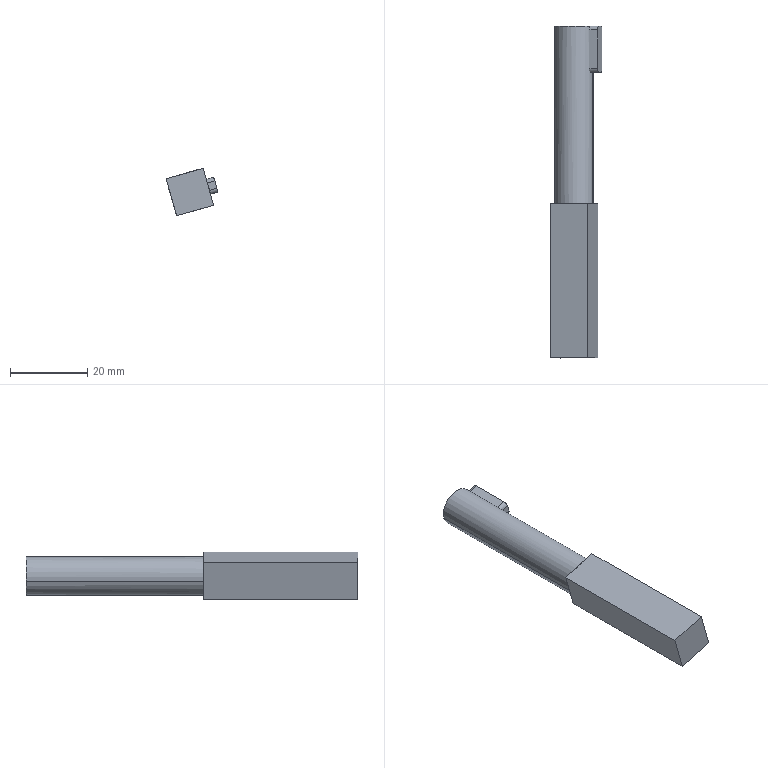Component | SolidWorks | DriveShaft2-2 | 1 solid | 20 faces | box 13.46 x 86 x 12.35 mm | volume 7713 mm3 | plane 14 | cylinder 6 | commonest cylinder face diameters 2 x4 10 x2
build123d program:
from build123d import *

# Parameters (mm, degrees)
SKETCH1_W                = 10
SKETCH1_H                = 10
BOSS_EXTRUDE1_DEPTH      = 40
SKETCH2_R                = 5
BOSS_EXTRUDE2_DEPTH      = 46
BOSS_EXTRUDE3_DEPTH      = 2
BOSS_EXTRUDE3_DEPTH_BACK = 6


with BuildPart() as part:
    # Sketch1 → Boss-Extrude1 (new body)
    with BuildSketch(Plane.XY):
        Rectangle(SKETCH1_W, SKETCH1_H)
    extrude(amount=BOSS_EXTRUDE1_DEPTH)

    # Sketch2 → Boss-Extrude2 (add)
    with BuildSketch(Plane(origin=(0, 0, 0), x_dir=(-1, 0, 0), z_dir=(0, 0, -1))):
        Circle(SKETCH2_R)
    extrude(amount=BOSS_EXTRUDE2_DEPTH)

    # Sketch3 → Boss-Extrude3 (add, two sides: drawn at the far end of the back side and taken through both)
    with BuildSketch(Plane(origin=(5, 0, 0), x_dir=(0, 0, -1), z_dir=(1, 0, 0)).offset(-BOSS_EXTRUDE3_DEPTH_BACK)):
        with BuildLine():
            Line((45, 2), (35, 2))
            ThreePointArc((35, 2), (34.293, 1.707), (34, 1))
            Line((34, 1), (34, -1))
            ThreePointArc((34, -1), (34.293, -1.707), (35, -2))
            Line((35, -2), (45, -2))
            ThreePointArc((45, -2), (45.707, -1.707), (46, -1))
            Line((46, -1), (46, 1))
            ThreePointArc((46, 1), (45.707, 1.707), (45, 2))
        make_face()
    extrude(amount=BOSS_EXTRUDE3_DEPTH + BOSS_EXTRUDE3_DEPTH_BACK)


solid = part.part

# Placed as in the assembly
solid = solid.moved(Location((-65.043, 476.747, 900.064), (90, 0, 15.845)))
STEP:
#1=COLOUR_RGB('',0.7922,0.8196,0.9333);
#2=FILL_AREA_STYLE_COLOUR('',#1);
#3=FILL_AREA_STYLE('',(#2));
#4=SURFACE_STYLE_FILL_AREA(#3);
#5=SURFACE_SIDE_STYLE('',(#4));
#6=SURFACE_STYLE_USAGE(.BOTH.,#5);
#7=PRESENTATION_STYLE_ASSIGNMENT((#6));
#8=CARTESIAN_POINT('',(-2.75,20.581,35.382));
#9=VERTEX_POINT('',#8);
#10=CARTESIAN_POINT('',(-2.386,20.581,35.526));
#11=VERTEX_POINT('',#10);
#12=CARTESIAN_POINT('',(-2.561,20.581,35.436));
#13=DIRECTION('',(-0.,1.,0.));
#14=DIRECTION('',(-0.962,0.,-0.273));
#15=AXIS2_PLACEMENT_3D('',#12,#13,#14);
#16=CIRCLE('',#15,0.1969);
#17=EDGE_CURVE('',#9,#11,#16,.T.);
#18=ORIENTED_EDGE('',*,*,#17,.F.);
#19=CARTESIAN_POINT('',(-2.75,18.77,35.382));
#20=VERTEX_POINT('',#19);
#21=CARTESIAN_POINT('',(-2.75,20.581,35.382));
#22=DIRECTION('',(0.,-1.,-0.));
#23=VECTOR('',#22,39.37);
#24=LINE('',#21,#23);
#25=EDGE_CURVE('',#9,#20,#24,.T.);
#26=ORIENTED_EDGE('',*,*,#25,.T.);
#27=CARTESIAN_POINT('',(-2.615,18.77,35.625));
#28=VERTEX_POINT('',#27);
#29=CARTESIAN_POINT('',(-2.561,18.77,35.436));
#30=DIRECTION('',(-0.,1.,0.));
#31=DIRECTION('',(-0.962,0.,-0.273));
#32=AXIS2_PLACEMENT_3D('',#29,#30,#31);
#33=CIRCLE('',#32,0.1969);
#34=EDGE_CURVE('',#20,#28,#33,.T.);
#35=ORIENTED_EDGE('',*,*,#34,.T.);
#36=CARTESIAN_POINT('',(-2.371,18.77,35.489));
#37=VERTEX_POINT('',#36);
#38=CARTESIAN_POINT('',(-2.561,18.77,35.436));
#39=DIRECTION('',(-0.,1.,0.));
#40=DIRECTION('',(-0.962,0.,-0.273));
#41=AXIS2_PLACEMENT_3D('',#38,#39,#40);
#42=CIRCLE('',#41,0.1969);
#43=EDGE_CURVE('',#28,#37,#42,.T.);
#44=ORIENTED_EDGE('',*,*,#43,.T.);
#45=CARTESIAN_POINT('',(-2.371,20.108,35.489));
#46=VERTEX_POINT('',#45);
#47=CARTESIAN_POINT('',(-2.371,20.581,35.489));
#48=DIRECTION('',(0.,-1.,-0.));
#49=VECTOR('',#48,39.37);
#50=LINE('',#47,#49);
#51=EDGE_CURVE('',#46,#37,#50,.T.);
#52=ORIENTED_EDGE('',*,*,#51,.F.);
#53=CARTESIAN_POINT('',(-2.386,20.108,35.526));
#54=VERTEX_POINT('',#53);
#55=CARTESIAN_POINT('',(-2.561,20.108,35.436));
#56=DIRECTION('',(0.,-1.,-0.));
#57=DIRECTION('',(0.962,0.,0.273));
#58=AXIS2_PLACEMENT_3D('',#55,#56,#57);
#59=CIRCLE('',#58,0.1969);
#60=EDGE_CURVE('',#46,#54,#59,.T.);
#61=ORIENTED_EDGE('',*,*,#60,.T.);
#62=CARTESIAN_POINT('',(-2.409,20.148,35.561));
#63=VERTEX_POINT('',#62);
#64=CARTESIAN_POINT('',(-2.386,20.108,35.526));
#65=CARTESIAN_POINT('',(-2.388,20.108,35.531));
#66=CARTESIAN_POINT('',(-2.391,20.109,35.535));
#67=CARTESIAN_POINT('',(-2.396,20.113,35.544));
#68=CARTESIAN_POINT('',(-2.399,20.116,35.547));
#69=CARTESIAN_POINT('',(-2.403,20.123,35.554));
#70=CARTESIAN_POINT('',(-2.405,20.127,35.556));
#71=CARTESIAN_POINT('',(-2.408,20.137,35.56));
#72=CARTESIAN_POINT('',(-2.409,20.142,35.561));
#73=CARTESIAN_POINT('',(-2.409,20.148,35.561));
#74=B_SPLINE_CURVE_WITH_KNOTS('',3,(#64,#65,#66,#67,#68,#69,#70,#71,#72,#73),.UNSPECIFIED.,.F.,.F.,(4,2,2,2,4),(0.00157,0.00197,0.00237,0.002769,0.003169),.UNSPECIFIED.);
#75=EDGE_CURVE('',#54,#63,#74,.T.);
#76=ORIENTED_EDGE('',*,*,#75,.T.);
#77=CARTESIAN_POINT('',(-2.409,20.541,35.561));
#78=VERTEX_POINT('',#77);
#79=CARTESIAN_POINT('',(-2.409,20.581,35.561));
#80=DIRECTION('',(-0.,1.,0.));
#81=VECTOR('',#80,39.37);
#82=LINE('',#79,#81);
#83=EDGE_CURVE('',#63,#78,#82,.T.);
#84=ORIENTED_EDGE('',*,*,#83,.T.);
#85=CARTESIAN_POINT('',(-2.386,20.581,35.526));
#86=CARTESIAN_POINT('',(-2.388,20.581,35.531));
#87=CARTESIAN_POINT('',(-2.391,20.58,35.535));
#88=CARTESIAN_POINT('',(-2.396,20.576,35.544));
#89=CARTESIAN_POINT('',(-2.399,20.573,35.547));
#90=CARTESIAN_POINT('',(-2.403,20.566,35.554));
#91=CARTESIAN_POINT('',(-2.405,20.561,35.556));
#92=CARTESIAN_POINT('',(-2.408,20.552,35.56));
#93=CARTESIAN_POINT('',(-2.409,20.547,35.561));
#94=CARTESIAN_POINT('',(-2.409,20.541,35.561));
#95=B_SPLINE_CURVE_WITH_KNOTS('',3,(#85,#86,#87,#88,#89,#90,#91,#92,#93,#94),.UNSPECIFIED.,.F.,.F.,(4,2,2,2,4),(0.,0.0003995,0.0007989,0.001198,0.001598),.UNSPECIFIED.);
#96=EDGE_CURVE('',#11,#78,#95,.T.);
#97=ORIENTED_EDGE('',*,*,#96,.F.);
#98=EDGE_LOOP('',(#18,#26,#35,#44,#52,#61,#76,#84,#97));
#99=FACE_OUTER_BOUND('',#98,.T.);
#100=CARTESIAN_POINT('',(-2.561,20.581,35.436));
#101=DIRECTION('',(0.,-1.,-0.));
#102=DIRECTION('',(0.962,0.,0.273));
#103=AXIS2_PLACEMENT_3D('',#100,#101,#102);
#104=CYLINDRICAL_SURFACE('',#103,0.1969);
#105=ADVANCED_FACE('',(#99),#104,.T.);
#106=ORIENTED_EDGE('',*,*,#25,.F.);
#107=CARTESIAN_POINT('',(-2.364,20.581,35.45));
#108=VERTEX_POINT('',#107);
#109=CARTESIAN_POINT('',(-2.561,20.581,35.436));
#110=DIRECTION('',(-0.,1.,0.));
#111=DIRECTION('',(-0.962,0.,-0.273));
#112=AXIS2_PLACEMENT_3D('',#109,#110,#111);
#113=CIRCLE('',#112,0.1969);
#114=EDGE_CURVE('',#108,#9,#113,.T.);
#115=ORIENTED_EDGE('',*,*,#114,.F.);
#116=CARTESIAN_POINT('',(-2.366,20.541,35.409));
#117=VERTEX_POINT('',#116);
#118=CARTESIAN_POINT('',(-2.364,20.581,35.45));
#119=CARTESIAN_POINT('',(-2.364,20.581,35.445));
#120=CARTESIAN_POINT('',(-2.364,20.58,35.44));
#121=CARTESIAN_POINT('',(-2.364,20.576,35.43));
#122=CARTESIAN_POINT('',(-2.364,20.573,35.425));
#123=CARTESIAN_POINT('',(-2.365,20.566,35.418));
#124=CARTESIAN_POINT('',(-2.365,20.561,35.415));
#125=CARTESIAN_POINT('',(-2.366,20.552,35.41));
#126=CARTESIAN_POINT('',(-2.366,20.546,35.409));
#127=CARTESIAN_POINT('',(-2.366,20.541,35.409));
#128=B_SPLINE_CURVE_WITH_KNOTS('',3,(#118,#119,#120,#121,#122,#123,#124,#125,#126,#127),.UNSPECIFIED.,.F.,.F.,(4,2,2,2,4),(0.,0.0003998,0.0007997,0.001199,0.001599),.UNSPECIFIED.);
#129=EDGE_CURVE('',#108,#117,#128,.T.);
#130=ORIENTED_EDGE('',*,*,#129,.T.);
#131=CARTESIAN_POINT('',(-2.366,20.148,35.409));
#132=VERTEX_POINT('',#131);
#133=CARTESIAN_POINT('',(-2.366,20.581,35.409));
#134=DIRECTION('',(0.,-1.,-0.));
#135=VECTOR('',#134,39.37);
#136=LINE('',#133,#135);
#137=EDGE_CURVE('',#117,#132,#136,.T.);
#138=ORIENTED_EDGE('',*,*,#137,.T.);
#139=CARTESIAN_POINT('',(-2.364,20.108,35.45));
#140=VERTEX_POINT('',#139);
#141=CARTESIAN_POINT('',(-2.366,20.148,35.409));
#142=CARTESIAN_POINT('',(-2.366,20.142,35.409));
#143=CARTESIAN_POINT('',(-2.366,20.137,35.41));
#144=CARTESIAN_POINT('',(-2.365,20.127,35.415));
#145=CARTESIAN_POINT('',(-2.365,20.123,35.418));
#146=CARTESIAN_POINT('',(-2.364,20.112,35.429));
#147=CARTESIAN_POINT('',(-2.364,20.108,35.44));
#148=CARTESIAN_POINT('',(-2.364,20.108,35.45));
#149=B_SPLINE_CURVE_WITH_KNOTS('',3,(#141,#142,#143,#144,#145,#146,#147,#148),.UNSPECIFIED.,.F.,.F.,(4,2,2,4),(0.003169,0.003569,0.003968,0.004767),.UNSPECIFIED.);
#150=EDGE_CURVE('',#132,#140,#149,.T.);
#151=ORIENTED_EDGE('',*,*,#150,.T.);
#152=CARTESIAN_POINT('',(-2.561,20.108,35.436));
#153=DIRECTION('',(0.,-1.,-0.));
#154=DIRECTION('',(0.962,0.,0.273));
#155=AXIS2_PLACEMENT_3D('',#152,#153,#154);
#156=CIRCLE('',#155,0.1969);
#157=EDGE_CURVE('',#140,#46,#156,.T.);
#158=ORIENTED_EDGE('',*,*,#157,.T.);
#159=ORIENTED_EDGE('',*,*,#51,.T.);
#160=CARTESIAN_POINT('',(-2.507,18.77,35.246));
#161=VERTEX_POINT('',#160);
#162=CARTESIAN_POINT('',(-2.561,18.77,35.436));
#163=DIRECTION('',(-0.,1.,0.));
#164=DIRECTION('',(-0.962,0.,-0.273));
#165=AXIS2_PLACEMENT_3D('',#162,#163,#164);
#166=CIRCLE('',#165,0.1969);
#167=EDGE_CURVE('',#37,#161,#166,.T.);
#168=ORIENTED_EDGE('',*,*,#167,.T.);
#169=CARTESIAN_POINT('',(-2.561,18.77,35.436));
#170=DIRECTION('',(-0.,1.,0.));
#171=DIRECTION('',(-0.962,0.,-0.273));
#172=AXIS2_PLACEMENT_3D('',#169,#170,#171);
#173=CIRCLE('',#172,0.1969);
#174=EDGE_CURVE('',#161,#20,#173,.T.);
#175=ORIENTED_EDGE('',*,*,#174,.T.);
#176=EDGE_LOOP('',(#106,#115,#130,#138,#151,#158,#159,#168,#175));
#177=FACE_OUTER_BOUND('',#176,.T.);
#178=CARTESIAN_POINT('',(-2.561,20.581,35.436));
#179=DIRECTION('',(0.,-1.,-0.));
#180=DIRECTION('',(0.962,0.,0.273));
#181=AXIS2_PLACEMENT_3D('',#178,#179,#180);
#182=CYLINDRICAL_SURFACE('',#181,0.1969);
#183=ADVANCED_FACE('',(#177),#182,.T.);
#184=ORIENTED_EDGE('',*,*,#34,.F.);
#185=CARTESIAN_POINT('',(-2.804,18.77,35.571));
#186=VERTEX_POINT('',#185);
#187=CARTESIAN_POINT('',(-2.696,18.77,35.192));
#188=DIRECTION('',(0.273,0.,-0.962));
#189=VECTOR('',#188,39.37);
#190=LINE('',#187,#189);
#191=EDGE_CURVE('',#186,#20,#190,.T.);
#192=ORIENTED_EDGE('',*,*,#191,.F.);
#193=CARTESIAN_POINT('',(-2.804,18.77,35.571));
#194=DIRECTION('',(-0.962,-0.,-0.273));
#195=VECTOR('',#194,39.37);
#196=LINE('',#193,#195);
#197=EDGE_CURVE('',#28,#186,#196,.T.);
#198=ORIENTED_EDGE('',*,*,#197,.F.);
#199=EDGE_LOOP('',(#184,#192,#198));
#200=FACE_OUTER_BOUND('',#199,.T.);
#201=CARTESIAN_POINT('',(-2.561,18.77,35.436));
#202=DIRECTION('',(-0.,1.,0.));
#203=DIRECTION('',(-0.962,-0.,-0.273));
#204=AXIS2_PLACEMENT_3D('',#201,#202,#203);
#205=PLANE('',#204);
#206=ADVANCED_FACE('',(#200),#205,.T.);
#207=ORIENTED_EDGE('',*,*,#43,.F.);
#208=CARTESIAN_POINT('',(-2.425,18.77,35.679));
#209=VERTEX_POINT('',#208);
#210=CARTESIAN_POINT('',(-2.804,18.77,35.571));
#211=DIRECTION('',(-0.962,-0.,-0.273));
#212=VECTOR('',#211,39.37);
#213=LINE('',#210,#212);
#214=EDGE_CURVE('',#209,#28,#213,.T.);
#215=ORIENTED_EDGE('',*,*,#214,.F.);
#216=CARTESIAN_POINT('',(-2.318,18.77,35.3));
#217=DIRECTION('',(-0.273,-0.,0.962));
#218=VECTOR('',#217,39.37);
#219=LINE('',#216,#218);
#220=EDGE_CURVE('',#37,#209,#219,.T.);
#221=ORIENTED_EDGE('',*,*,#220,.F.);
#222=EDGE_LOOP('',(#207,#215,#221));
#223=FACE_OUTER_BOUND('',#222,.T.);
#224=CARTESIAN_POINT('',(-2.561,18.77,35.436));
#225=DIRECTION('',(-0.,1.,0.));
#226=DIRECTION('',(-0.962,-0.,-0.273));
#227=AXIS2_PLACEMENT_3D('',#224,#225,#226);
#228=PLANE('',#227);
#229=ADVANCED_FACE('',(#223),#228,.T.);
#230=ORIENTED_EDGE('',*,*,#167,.F.);
#231=CARTESIAN_POINT('',(-2.318,18.77,35.3));
#232=VERTEX_POINT('',#231);
#233=CARTESIAN_POINT('',(-2.318,18.77,35.3));
#234=DIRECTION('',(-0.273,-0.,0.962));
#235=VECTOR('',#234,39.37);
#236=LINE('',#233,#235);
#237=EDGE_CURVE('',#232,#37,#236,.T.);
#238=ORIENTED_EDGE('',*,*,#237,.F.);
#239=CARTESIAN_POINT('',(-2.696,18.77,35.192));
#240=DIRECTION('',(0.962,0.,0.273));
#241=VECTOR('',#240,39.37);
#242=LINE('',#239,#241);
#243=EDGE_CURVE('',#161,#232,#242,.T.);
#244=ORIENTED_EDGE('',*,*,#243,.F.);
#245=EDGE_LOOP('',(#230,#238,#244));
#246=FACE_OUTER_BOUND('',#245,.T.);
#247=CARTESIAN_POINT('',(-2.561,18.77,35.436));
#248=DIRECTION('',(-0.,1.,0.));
#249=DIRECTION('',(-0.962,-0.,-0.273));
#250=AXIS2_PLACEMENT_3D('',#247,#248,#249);
#251=PLANE('',#250);
#252=ADVANCED_FACE('',(#246),#251,.T.);
#253=ORIENTED_EDGE('',*,*,#237,.T.);
#254=ORIENTED_EDGE('',*,*,#220,.T.);
#255=CARTESIAN_POINT('',(-2.425,17.195,35.679));
#256=VERTEX_POINT('',#255);
#257=CARTESIAN_POINT('',(-2.425,17.195,35.679));
#258=DIRECTION('',(-0.,1.,0.));
#259=VECTOR('',#258,39.37);
#260=LINE('',#257,#259);
#261=EDGE_CURVE('',#256,#209,#260,.T.);
#262=ORIENTED_EDGE('',*,*,#261,.F.);
#263=CARTESIAN_POINT('',(-2.318,17.195,35.3));
#264=VERTEX_POINT('',#263);
#265=CARTESIAN_POINT('',(-2.318,17.195,35.3));
#266=DIRECTION('',(-0.273,-0.,0.962));
#267=VECTOR('',#266,39.37);
#268=LINE('',#265,#267);
#269=EDGE_CURVE('',#264,#256,#268,.T.);
#270=ORIENTED_EDGE('',*,*,#269,.F.);
#271=CARTESIAN_POINT('',(-2.318,17.195,35.3));
#272=DIRECTION('',(-0.,1.,0.));
#273=VECTOR('',#272,39.37);
#274=LINE('',#271,#273);
#275=EDGE_CURVE('',#264,#232,#274,.T.);
#276=ORIENTED_EDGE('',*,*,#275,.T.);
#277=EDGE_LOOP('',(#253,#254,#262,#270,#276));
#278=FACE_OUTER_BOUND('',#277,.T.);
#279=CARTESIAN_POINT('',(-2.318,17.195,35.3));
#280=DIRECTION('',(-0.962,-0.,-0.273));
#281=DIRECTION('',(0.,-1.,-0.));
#282=AXIS2_PLACEMENT_3D('',#279,#280,#281);
#283=PLANE('',#282);
#284=ADVANCED_FACE('',(#278),#283,.F.);
#285=ORIENTED_EDGE('',*,*,#214,.T.);
#286=ORIENTED_EDGE('',*,*,#197,.T.);
#287=CARTESIAN_POINT('',(-2.804,17.195,35.571));
#288=VERTEX_POINT('',#287);
#289=CARTESIAN_POINT('',(-2.804,17.195,35.571));
#290=DIRECTION('',(-0.,1.,0.));
#291=VECTOR('',#290,39.37);
#292=LINE('',#289,#291);
#293=EDGE_CURVE('',#288,#186,#292,.T.);
#294=ORIENTED_EDGE('',*,*,#293,.F.);
#295=CARTESIAN_POINT('',(-2.804,17.195,35.571));
#296=DIRECTION('',(-0.962,-0.,-0.273));
#297=VECTOR('',#296,39.37);
#298=LINE('',#295,#297);
#299=EDGE_CURVE('',#256,#288,#298,.T.);
#300=ORIENTED_EDGE('',*,*,#299,.F.);
#301=ORIENTED_EDGE('',*,*,#261,.T.);
#302=EDGE_LOOP('',(#285,#286,#294,#300,#301));
#303=FACE_OUTER_BOUND('',#302,.T.);
#304=CARTESIAN_POINT('',(-2.804,17.195,35.571));
#305=DIRECTION('',(0.273,0.,-0.962));
#306=DIRECTION('',(-0.,1.,0.));
#307=AXIS2_PLACEMENT_3D('',#304,#305,#306);
#308=PLANE('',#307);
#309=ADVANCED_FACE('',(#303),#308,.F.);
#310=ORIENTED_EDGE('',*,*,#191,.T.);
#311=CARTESIAN_POINT('',(-2.696,18.77,35.192));
#312=VERTEX_POINT('',#311);
#313=CARTESIAN_POINT('',(-2.696,18.77,35.192));
#314=DIRECTION('',(0.273,0.,-0.962));
#315=VECTOR('',#314,39.37);
#316=LINE('',#313,#315);
#317=EDGE_CURVE('',#20,#312,#316,.T.);
#318=ORIENTED_EDGE('',*,*,#317,.T.);
#319=CARTESIAN_POINT('',(-2.696,17.195,35.192));
#320=VERTEX_POINT('',#319);
#321=CARTESIAN_POINT('',(-2.696,17.195,35.192));
#322=DIRECTION('',(-0.,1.,0.));
#323=VECTOR('',#322,39.37);
#324=LINE('',#321,#323);
#325=EDGE_CURVE('',#320,#312,#324,.T.);
#326=ORIENTED_EDGE('',*,*,#325,.F.);
#327=CARTESIAN_POINT('',(-2.696,17.195,35.192));
#328=DIRECTION('',(0.273,0.,-0.962));
#329=VECTOR('',#328,39.37);
#330=LINE('',#327,#329);
#331=EDGE_CURVE('',#288,#320,#330,.T.);
#332=ORIENTED_EDGE('',*,*,#331,.F.);
#333=ORIENTED_EDGE('',*,*,#293,.T.);
#334=EDGE_LOOP('',(#310,#318,#326,#332,#333));
#335=FACE_OUTER_BOUND('',#334,.T.);
#336=CARTESIAN_POINT('',(-2.696,17.195,35.192));
#337=DIRECTION('',(0.962,0.,0.273));
#338=DIRECTION('',(-0.,1.,0.));
#339=AXIS2_PLACEMENT_3D('',#336,#337,#338);
#340=PLANE('',#339);
#341=ADVANCED_FACE('',(#335),#340,.F.);
#342=CARTESIAN_POINT('',(-2.696,18.77,35.192));
#343=DIRECTION('',(0.962,0.,0.273));
#344=VECTOR('',#343,39.37);
#345=LINE('',#342,#344);
#346=EDGE_CURVE('',#312,#161,#345,.T.);
#347=ORIENTED_EDGE('',*,*,#346,.T.);
#348=ORIENTED_EDGE('',*,*,#243,.T.);
#349=ORIENTED_EDGE('',*,*,#275,.F.);
#350=CARTESIAN_POINT('',(-2.696,17.195,35.192));
#351=DIRECTION('',(0.962,0.,0.273));
#352=VECTOR('',#351,39.37);
#353=LINE('',#350,#352);
#354=EDGE_CURVE('',#320,#264,#353,.T.);
#355=ORIENTED_EDGE('',*,*,#354,.F.);
#356=ORIENTED_EDGE('',*,*,#325,.T.);
#357=EDGE_LOOP('',(#347,#348,#349,#355,#356));
#358=FACE_OUTER_BOUND('',#357,.T.);
#359=CARTESIAN_POINT('',(-2.696,17.195,35.192));
#360=DIRECTION('',(-0.273,-0.,0.962));
#361=DIRECTION('',(0.,-1.,-0.));
#362=AXIS2_PLACEMENT_3D('',#359,#360,#361);
#363=PLANE('',#362);
#364=ADVANCED_FACE('',(#358),#363,.F.);
#365=ORIENTED_EDGE('',*,*,#269,.T.);
#366=ORIENTED_EDGE('',*,*,#299,.T.);
#367=ORIENTED_EDGE('',*,*,#331,.T.);
#368=ORIENTED_EDGE('',*,*,#354,.T.);
#369=EDGE_LOOP('',(#365,#366,#367,#368));
#370=FACE_OUTER_BOUND('',#369,.T.);
#371=CARTESIAN_POINT('',(-2.561,17.195,35.436));
#372=DIRECTION('',(-0.,1.,0.));
#373=DIRECTION('',(-0.962,-0.,-0.273));
#374=AXIS2_PLACEMENT_3D('',#371,#372,#373);
#375=PLANE('',#374);
#376=ADVANCED_FACE('',(#370),#375,.F.);
#377=ORIENTED_EDGE('',*,*,#174,.F.);
#378=ORIENTED_EDGE('',*,*,#346,.F.);
#379=ORIENTED_EDGE('',*,*,#317,.F.);
#380=EDGE_LOOP('',(#377,#378,#379));
#381=FACE_OUTER_BOUND('',#380,.T.);
#382=CARTESIAN_POINT('',(-2.561,18.77,35.436));
#383=DIRECTION('',(-0.,1.,0.));
#384=DIRECTION('',(-0.962,-0.,-0.273));
#385=AXIS2_PLACEMENT_3D('',#382,#383,#384);
#386=PLANE('',#385);
#387=ADVANCED_FACE('',(#381),#386,.T.);
#388=ORIENTED_EDGE('',*,*,#114,.T.);
#389=ORIENTED_EDGE('',*,*,#17,.T.);
#390=CARTESIAN_POINT('',(-2.306,20.581,35.549));
#391=VERTEX_POINT('',#390);
#392=CARTESIAN_POINT('',(-2.609,20.581,35.463));
#393=DIRECTION('',(0.962,0.,0.273));
#394=VECTOR('',#393,39.37);
#395=LINE('',#392,#394);
#396=EDGE_CURVE('',#11,#391,#395,.T.);
#397=ORIENTED_EDGE('',*,*,#396,.T.);
#398=CARTESIAN_POINT('',(-2.285,20.581,35.473));
#399=VERTEX_POINT('',#398);
#400=CARTESIAN_POINT('',(-2.285,20.581,35.473));
#401=DIRECTION('',(-0.273,-0.,0.962));
#402=VECTOR('',#401,39.37);
#403=LINE('',#400,#402);
#404=EDGE_CURVE('',#399,#391,#403,.T.);
#405=ORIENTED_EDGE('',*,*,#404,.F.);
#406=CARTESIAN_POINT('',(-2.588,20.581,35.387));
#407=DIRECTION('',(0.962,0.,0.273));
#408=VECTOR('',#407,39.37);
#409=LINE('',#406,#408);
#410=EDGE_CURVE('',#108,#399,#409,.T.);
#411=ORIENTED_EDGE('',*,*,#410,.F.);
#412=EDGE_LOOP('',(#388,#389,#397,#405,#411));
#413=FACE_OUTER_BOUND('',#412,.T.);
#414=CARTESIAN_POINT('',(-2.561,20.581,35.436));
#415=DIRECTION('',(-0.,1.,0.));
#416=DIRECTION('',(-0.962,-0.,-0.273));
#417=AXIS2_PLACEMENT_3D('',#414,#415,#416);
#418=PLANE('',#417);
#419=ADVANCED_FACE('',(#413),#418,.T.);
#420=ORIENTED_EDGE('',*,*,#137,.F.);
#421=CARTESIAN_POINT('',(-2.274,20.541,35.435));
#422=VERTEX_POINT('',#421);
#423=CARTESIAN_POINT('',(-2.577,20.541,35.349));
#424=DIRECTION('',(0.962,0.,0.273));
#425=VECTOR('',#424,39.37);
#426=LINE('',#423,#425);
#427=EDGE_CURVE('',#117,#422,#426,.T.);
#428=ORIENTED_EDGE('',*,*,#427,.T.);
#429=CARTESIAN_POINT('',(-2.274,20.148,35.435));
#430=VERTEX_POINT('',#429);
#431=CARTESIAN_POINT('',(-2.274,20.148,35.435));
#432=DIRECTION('',(-0.,1.,0.));
#433=VECTOR('',#432,39.37);
#434=LINE('',#431,#433);
#435=EDGE_CURVE('',#430,#422,#434,.T.);
#436=ORIENTED_EDGE('',*,*,#435,.F.);
#437=CARTESIAN_POINT('',(-2.577,20.148,35.349));
#438=DIRECTION('',(0.962,0.,0.273));
#439=VECTOR('',#438,39.37);
#440=LINE('',#437,#439);
#441=EDGE_CURVE('',#132,#430,#440,.T.);
#442=ORIENTED_EDGE('',*,*,#441,.F.);
#443=EDGE_LOOP('',(#420,#428,#436,#442));
#444=FACE_OUTER_BOUND('',#443,.T.);
#445=CARTESIAN_POINT('',(-2.577,20.148,35.349));
#446=DIRECTION('',(0.273,0.,-0.962));
#447=DIRECTION('',(-0.,1.,0.));
#448=AXIS2_PLACEMENT_3D('',#445,#446,#447);
#449=PLANE('',#448);
#450=ADVANCED_FACE('',(#444),#449,.T.);
#451=ORIENTED_EDGE('',*,*,#150,.F.);
#452=ORIENTED_EDGE('',*,*,#441,.T.);
#453=CARTESIAN_POINT('',(-2.285,20.108,35.473));
#454=VERTEX_POINT('',#453);
#455=CARTESIAN_POINT('',(-2.285,20.148,35.473));
#456=DIRECTION('',(0.962,0.,0.273));
#457=DIRECTION('',(0.,1.,0.));
#458=AXIS2_PLACEMENT_3D('',#455,#456,#457);
#459=CIRCLE('',#458,0.03937);
#460=EDGE_CURVE('',#454,#430,#459,.T.);
#461=ORIENTED_EDGE('',*,*,#460,.F.);
#462=CARTESIAN_POINT('',(-2.588,20.108,35.387));
#463=DIRECTION('',(0.962,0.,0.273));
#464=VECTOR('',#463,39.37);
#465=LINE('',#462,#464);
#466=EDGE_CURVE('',#140,#454,#465,.T.);
#467=ORIENTED_EDGE('',*,*,#466,.F.);
#468=EDGE_LOOP('',(#451,#452,#461,#467));
#469=FACE_OUTER_BOUND('',#468,.T.);
#470=CARTESIAN_POINT('',(-2.588,20.148,35.387));
#471=DIRECTION('',(0.962,0.,0.273));
#472=DIRECTION('',(0.,1.,0.));
#473=AXIS2_PLACEMENT_3D('',#470,#471,#472);
#474=CYLINDRICAL_SURFACE('',#473,0.03937);
#475=ADVANCED_FACE('',(#469),#474,.T.);
#476=ORIENTED_EDGE('',*,*,#75,.F.);
#477=CARTESIAN_POINT('',(-2.306,20.108,35.549));
#478=VERTEX_POINT('',#477);
#479=CARTESIAN_POINT('',(-2.609,20.108,35.463));
#480=DIRECTION('',(0.962,0.,0.273));
#481=VECTOR('',#480,39.37);
#482=LINE('',#479,#481);
#483=EDGE_CURVE('',#54,#478,#482,.T.);
#484=ORIENTED_EDGE('',*,*,#483,.T.);
#485=CARTESIAN_POINT('',(-2.317,20.148,35.587));
#486=VERTEX_POINT('',#485);
#487=CARTESIAN_POINT('',(-2.306,20.148,35.549));
#488=DIRECTION('',(0.962,0.,0.273));
#489=DIRECTION('',(0.,1.,0.));
#490=AXIS2_PLACEMENT_3D('',#487,#488,#489);
#491=CIRCLE('',#490,0.03937);
#492=EDGE_CURVE('',#486,#478,#491,.T.);
#493=ORIENTED_EDGE('',*,*,#492,.F.);
#494=CARTESIAN_POINT('',(-2.62,20.148,35.501));
#495=DIRECTION('',(0.962,0.,0.273));
#496=VECTOR('',#495,39.37);
#497=LINE('',#494,#496);
#498=EDGE_CURVE('',#63,#486,#497,.T.);
#499=ORIENTED_EDGE('',*,*,#498,.F.);
#500=EDGE_LOOP('',(#476,#484,#493,#499));
#501=FACE_OUTER_BOUND('',#500,.T.);
#502=CARTESIAN_POINT('',(-2.609,20.148,35.463));
#503=DIRECTION('',(0.962,0.,0.273));
#504=DIRECTION('',(0.,1.,0.));
#505=AXIS2_PLACEMENT_3D('',#502,#503,#504);
#506=CYLINDRICAL_SURFACE('',#505,0.03937);
#507=ADVANCED_FACE('',(#501),#506,.T.);
#508=ORIENTED_EDGE('',*,*,#83,.F.);
#509=ORIENTED_EDGE('',*,*,#498,.T.);
#510=CARTESIAN_POINT('',(-2.317,20.541,35.587));
#511=VERTEX_POINT('',#510);
#512=CARTESIAN_POINT('',(-2.317,20.541,35.587));
#513=DIRECTION('',(0.,-1.,-0.));
#514=VECTOR('',#513,39.37);
#515=LINE('',#512,#514);
#516=EDGE_CURVE('',#511,#486,#515,.T.);
#517=ORIENTED_EDGE('',*,*,#516,.F.);
#518=CARTESIAN_POINT('',(-2.62,20.541,35.501));
#519=DIRECTION('',(0.962,0.,0.273));
#520=VECTOR('',#519,39.37);
#521=LINE('',#518,#520);
#522=EDGE_CURVE('',#78,#511,#521,.T.);
#523=ORIENTED_EDGE('',*,*,#522,.F.);
#524=EDGE_LOOP('',(#508,#509,#517,#523));
#525=FACE_OUTER_BOUND('',#524,.T.);
#526=CARTESIAN_POINT('',(-2.62,20.541,35.501));
#527=DIRECTION('',(-0.273,-0.,0.962));
#528=DIRECTION('',(0.,-1.,-0.));
#529=AXIS2_PLACEMENT_3D('',#526,#527,#528);
#530=PLANE('',#529);
#531=ADVANCED_FACE('',(#525),#530,.T.);
#532=ORIENTED_EDGE('',*,*,#396,.F.);
#533=ORIENTED_EDGE('',*,*,#96,.T.);
#534=ORIENTED_EDGE('',*,*,#522,.T.);
#535=CARTESIAN_POINT('',(-2.306,20.541,35.549));
#536=DIRECTION('',(-0.962,-0.,-0.273));
#537=DIRECTION('',(0.,-1.,0.));
#538=AXIS2_PLACEMENT_3D('',#535,#536,#537);
#539=CIRCLE('',#538,0.03937);
#540=EDGE_CURVE('',#511,#391,#539,.T.);
#541=ORIENTED_EDGE('',*,*,#540,.T.);
#542=EDGE_LOOP('',(#532,#533,#534,#541));
#543=FACE_OUTER_BOUND('',#542,.T.);
#544=CARTESIAN_POINT('',(-2.609,20.541,35.463));
#545=DIRECTION('',(0.962,0.,0.273));
#546=DIRECTION('',(0.,1.,0.));
#547=AXIS2_PLACEMENT_3D('',#544,#545,#546);
#548=CYLINDRICAL_SURFACE('',#547,0.03937);
#549=ADVANCED_FACE('',(#543),#548,.T.);
#550=ORIENTED_EDGE('',*,*,#129,.F.);
#551=ORIENTED_EDGE('',*,*,#410,.T.);
#552=CARTESIAN_POINT('',(-2.285,20.541,35.473));
#553=DIRECTION('',(0.962,0.,0.273));
#554=DIRECTION('',(0.,1.,0.));
#555=AXIS2_PLACEMENT_3D('',#552,#553,#554);
#556=CIRCLE('',#555,0.03937);
#557=EDGE_CURVE('',#422,#399,#556,.T.);
#558=ORIENTED_EDGE('',*,*,#557,.F.);
#559=ORIENTED_EDGE('',*,*,#427,.F.);
#560=EDGE_LOOP('',(#550,#551,#558,#559));
#561=FACE_OUTER_BOUND('',#560,.T.);
#562=CARTESIAN_POINT('',(-2.588,20.541,35.387));
#563=DIRECTION('',(0.962,0.,0.273));
#564=DIRECTION('',(0.,1.,0.));
#565=AXIS2_PLACEMENT_3D('',#562,#563,#564);
#566=CYLINDRICAL_SURFACE('',#565,0.03937);
#567=ADVANCED_FACE('',(#561),#566,.T.);
#568=ORIENTED_EDGE('',*,*,#157,.F.);
#569=ORIENTED_EDGE('',*,*,#466,.T.);
#570=CARTESIAN_POINT('',(-2.306,20.108,35.549));
#571=DIRECTION('',(0.273,0.,-0.962));
#572=VECTOR('',#571,39.37);
#573=LINE('',#570,#572);
#574=EDGE_CURVE('',#478,#454,#573,.T.);
#575=ORIENTED_EDGE('',*,*,#574,.F.);
#576=ORIENTED_EDGE('',*,*,#483,.F.);
#577=ORIENTED_EDGE('',*,*,#60,.F.);
#578=EDGE_LOOP('',(#568,#569,#575,#576,#577));
#579=FACE_OUTER_BOUND('',#578,.T.);
#580=CARTESIAN_POINT('',(-2.609,20.108,35.463));
#581=DIRECTION('',(0.,-1.,-0.));
#582=DIRECTION('',(0.962,0.,0.273));
#583=AXIS2_PLACEMENT_3D('',#580,#581,#582);
#584=PLANE('',#583);
#585=ADVANCED_FACE('',(#579),#584,.T.);
#586=ORIENTED_EDGE('',*,*,#540,.F.);
#587=ORIENTED_EDGE('',*,*,#516,.T.);
#588=ORIENTED_EDGE('',*,*,#492,.T.);
#589=ORIENTED_EDGE('',*,*,#574,.T.);
#590=ORIENTED_EDGE('',*,*,#460,.T.);
#591=ORIENTED_EDGE('',*,*,#435,.T.);
#592=ORIENTED_EDGE('',*,*,#557,.T.);
#593=ORIENTED_EDGE('',*,*,#404,.T.);
#594=EDGE_LOOP('',(#586,#587,#588,#589,#590,#591,#592,#593));
#595=FACE_OUTER_BOUND('',#594,.T.);
#596=CARTESIAN_POINT('',(-2.306,20.541,35.549));
#597=DIRECTION('',(-0.962,-0.,-0.273));
#598=DIRECTION('',(0.,-1.,-0.));
#599=AXIS2_PLACEMENT_3D('',#596,#597,#598);
#600=PLANE('',#599);
#601=ADVANCED_FACE('',(#595),#600,.F.);
#602=CLOSED_SHELL('',(#105,#183,#206,#229,#252,#284,#309,#341,#364,#376,#387,#419,#450,#475,#507,#531,#549,#567,#585,#601));
#603=MANIFOLD_SOLID_BREP('',#602);
#604=STYLED_ITEM('',(#7),#603);
#605=(LENGTH_UNIT()NAMED_UNIT(*)SI_UNIT($,.METRE.));
#606=LENGTH_MEASURE_WITH_UNIT(LENGTH_MEASURE(0.0254),#605);
#607=DIMENSIONAL_EXPONENTS(1.,0.,0.,0.,0.,0.,0.);
#608=(CONVERSION_BASED_UNIT('',#606)LENGTH_UNIT()NAMED_UNIT(#607));
#609=UNCERTAINTY_MEASURE_WITH_UNIT(LENGTH_MEASURE(0.00001),#608,'','');
#610=(NAMED_UNIT(*)PLANE_ANGLE_UNIT()SI_UNIT($,.RADIAN.));
#611=(NAMED_UNIT(*)SI_UNIT($,.STERADIAN.)SOLID_ANGLE_UNIT());
#612=(GEOMETRIC_REPRESENTATION_CONTEXT(3)GLOBAL_UNCERTAINTY_ASSIGNED_CONTEXT((#609))GLOBAL_UNIT_ASSIGNED_CONTEXT((#608,#610,#611))REPRESENTATION_CONTEXT('',''));
#613=MECHANICAL_DESIGN_GEOMETRIC_PRESENTATION_REPRESENTATION('',(#604),#612);
#614=CARTESIAN_POINT('',(0.,0.,0.));
#615=DIRECTION('',(0.,0.,1.));
#616=DIRECTION('',(1.,0.,0.));
#617=AXIS2_PLACEMENT_3D('',#614,#615,#616);
#618=(LENGTH_UNIT()NAMED_UNIT(*)SI_UNIT($,.METRE.));
#619=LENGTH_MEASURE_WITH_UNIT(LENGTH_MEASURE(0.0254),#618);
#620=DIMENSIONAL_EXPONENTS(1.,0.,0.,0.,0.,0.,0.);
#621=(CONVERSION_BASED_UNIT('',#619)LENGTH_UNIT()NAMED_UNIT(#620));
#622=UNCERTAINTY_MEASURE_WITH_UNIT(LENGTH_MEASURE(0.00001),#621,'','');
#623=(NAMED_UNIT(*)PLANE_ANGLE_UNIT()SI_UNIT($,.RADIAN.));
#624=(NAMED_UNIT(*)SI_UNIT($,.STERADIAN.)SOLID_ANGLE_UNIT());
#625=(GEOMETRIC_REPRESENTATION_CONTEXT(3)GLOBAL_UNCERTAINTY_ASSIGNED_CONTEXT((#622))GLOBAL_UNIT_ASSIGNED_CONTEXT((#621,#623,#624))REPRESENTATION_CONTEXT('',''));
#626=ADVANCED_BREP_SHAPE_REPRESENTATION('',(#603,#617),#625);
#627=PRESENTATION_LAYER_ASSIGNMENT('','',(#604));